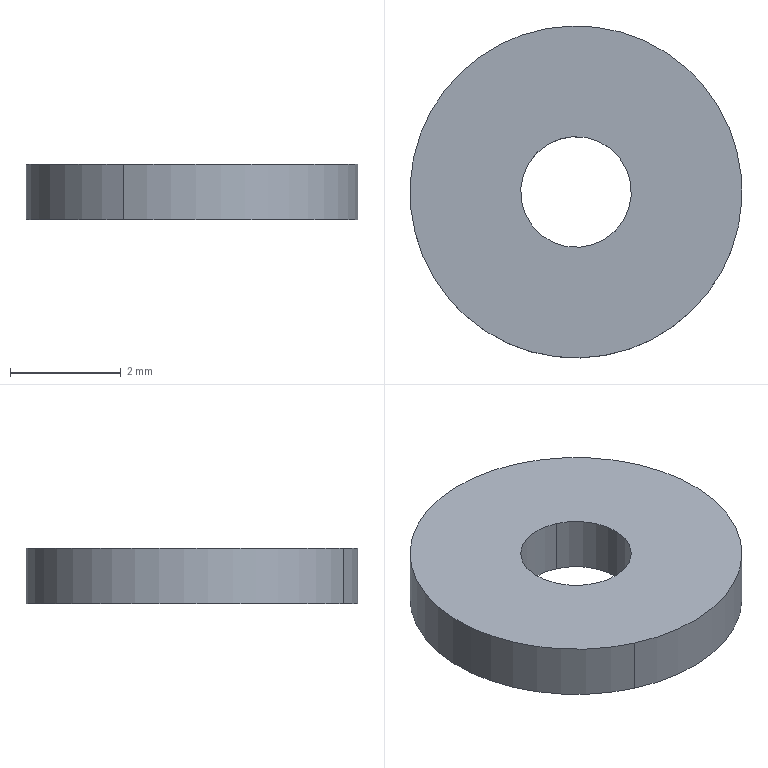Component | SolidWorks | Part28^Assembly1-2 | 1 solid | 6 faces | box 6 x 6 x 1 mm | volume 25 mm3 | cylinder 4 | plane 2 | commonest cylinder face diameters 2 x2 6 x2
STEP:
#1=COLOUR_RGB('',0.7922,0.8196,0.9333);
#2=FILL_AREA_STYLE_COLOUR('',#1);
#3=FILL_AREA_STYLE('',(#2));
#4=SURFACE_STYLE_FILL_AREA(#3);
#5=SURFACE_SIDE_STYLE('',(#4));
#6=SURFACE_STYLE_USAGE(.BOTH.,#5);
#7=PRESENTATION_STYLE_ASSIGNMENT((#6));
#8=CARTESIAN_POINT('',(0.5083,-0.1019,0.1575));
#9=VERTEX_POINT('',#8);
#10=CARTESIAN_POINT('',(0.4759,-0.1737,0.1575));
#11=VERTEX_POINT('',#10);
#12=CARTESIAN_POINT('',(0.4921,-0.1378,0.1575));
#13=DIRECTION('',(-0.,-0.,1.));
#14=DIRECTION('',(-0.412,-0.9112,-0.));
#15=AXIS2_PLACEMENT_3D('',#12,#13,#14);
#16=CIRCLE('',#15,0.03937);
#17=EDGE_CURVE('',#9,#11,#16,.T.);
#18=ORIENTED_EDGE('',*,*,#17,.T.);
#19=CARTESIAN_POINT('',(0.4759,-0.1737,0.1181));
#20=VERTEX_POINT('',#19);
#21=CARTESIAN_POINT('',(0.4759,-0.1737,0.1575));
#22=DIRECTION('',(0.,0.,-1.));
#23=VECTOR('',#22,39.37);
#24=LINE('',#21,#23);
#25=EDGE_CURVE('',#11,#20,#24,.T.);
#26=ORIENTED_EDGE('',*,*,#25,.T.);
#27=CARTESIAN_POINT('',(0.5083,-0.1019,0.1181));
#28=VERTEX_POINT('',#27);
#29=CARTESIAN_POINT('',(0.4921,-0.1378,0.1181));
#30=DIRECTION('',(-0.,-0.,1.));
#31=DIRECTION('',(-0.412,-0.9112,-0.));
#32=AXIS2_PLACEMENT_3D('',#29,#30,#31);
#33=CIRCLE('',#32,0.03937);
#34=EDGE_CURVE('',#28,#20,#33,.T.);
#35=ORIENTED_EDGE('',*,*,#34,.F.);
#36=CARTESIAN_POINT('',(0.5083,-0.1019,0.1575));
#37=DIRECTION('',(0.,0.,-1.));
#38=VECTOR('',#37,39.37);
#39=LINE('',#36,#38);
#40=EDGE_CURVE('',#9,#28,#39,.T.);
#41=ORIENTED_EDGE('',*,*,#40,.F.);
#42=EDGE_LOOP('',(#18,#26,#35,#41));
#43=FACE_OUTER_BOUND('',#42,.T.);
#44=CARTESIAN_POINT('',(0.4921,-0.1378,0.1575));
#45=DIRECTION('',(0.,0.,-1.));
#46=DIRECTION('',(0.412,0.9112,0.));
#47=AXIS2_PLACEMENT_3D('',#44,#45,#46);
#48=CYLINDRICAL_SURFACE('',#47,0.03937);
#49=ADVANCED_FACE('',(#43),#48,.F.);
#50=CARTESIAN_POINT('',(0.4435,-0.2454,0.1575));
#51=VERTEX_POINT('',#50);
#52=CARTESIAN_POINT('',(0.5408,-0.03017,0.1575));
#53=VERTEX_POINT('',#52);
#54=CARTESIAN_POINT('',(0.4921,-0.1378,0.1575));
#55=DIRECTION('',(-0.,-0.,1.));
#56=DIRECTION('',(-0.412,-0.9112,-0.));
#57=AXIS2_PLACEMENT_3D('',#54,#55,#56);
#58=CIRCLE('',#57,0.1181);
#59=EDGE_CURVE('',#51,#53,#58,.T.);
#60=ORIENTED_EDGE('',*,*,#59,.F.);
#61=CARTESIAN_POINT('',(0.4435,-0.2454,0.1181));
#62=VERTEX_POINT('',#61);
#63=CARTESIAN_POINT('',(0.4435,-0.2454,0.1575));
#64=DIRECTION('',(0.,0.,-1.));
#65=VECTOR('',#64,39.37);
#66=LINE('',#63,#65);
#67=EDGE_CURVE('',#51,#62,#66,.T.);
#68=ORIENTED_EDGE('',*,*,#67,.T.);
#69=CARTESIAN_POINT('',(0.5408,-0.03017,0.1181));
#70=VERTEX_POINT('',#69);
#71=CARTESIAN_POINT('',(0.4921,-0.1378,0.1181));
#72=DIRECTION('',(-0.,-0.,1.));
#73=DIRECTION('',(-0.412,-0.9112,-0.));
#74=AXIS2_PLACEMENT_3D('',#71,#72,#73);
#75=CIRCLE('',#74,0.1181);
#76=EDGE_CURVE('',#62,#70,#75,.T.);
#77=ORIENTED_EDGE('',*,*,#76,.T.);
#78=CARTESIAN_POINT('',(0.5408,-0.03017,0.1575));
#79=DIRECTION('',(0.,0.,-1.));
#80=VECTOR('',#79,39.37);
#81=LINE('',#78,#80);
#82=EDGE_CURVE('',#53,#70,#81,.T.);
#83=ORIENTED_EDGE('',*,*,#82,.F.);
#84=EDGE_LOOP('',(#60,#68,#77,#83));
#85=FACE_OUTER_BOUND('',#84,.T.);
#86=CARTESIAN_POINT('',(0.4921,-0.1378,0.1575));
#87=DIRECTION('',(0.,0.,-1.));
#88=DIRECTION('',(0.412,0.9112,0.));
#89=AXIS2_PLACEMENT_3D('',#86,#87,#88);
#90=CYLINDRICAL_SURFACE('',#89,0.1181);
#91=ADVANCED_FACE('',(#85),#90,.T.);
#92=CARTESIAN_POINT('',(0.4921,-0.1378,0.1575));
#93=DIRECTION('',(-0.,-0.,1.));
#94=DIRECTION('',(-0.412,-0.9112,-0.));
#95=AXIS2_PLACEMENT_3D('',#92,#93,#94);
#96=CIRCLE('',#95,0.1181);
#97=EDGE_CURVE('',#53,#51,#96,.T.);
#98=ORIENTED_EDGE('',*,*,#97,.T.);
#99=ORIENTED_EDGE('',*,*,#59,.T.);
#100=EDGE_LOOP('',(#98,#99));
#101=FACE_OUTER_BOUND('',#100,.T.);
#102=ORIENTED_EDGE('',*,*,#17,.F.);
#103=CARTESIAN_POINT('',(0.4921,-0.1378,0.1575));
#104=DIRECTION('',(-0.,-0.,1.));
#105=DIRECTION('',(-0.412,-0.9112,-0.));
#106=AXIS2_PLACEMENT_3D('',#103,#104,#105);
#107=CIRCLE('',#106,0.03937);
#108=EDGE_CURVE('',#11,#9,#107,.T.);
#109=ORIENTED_EDGE('',*,*,#108,.F.);
#110=EDGE_LOOP('',(#102,#109));
#111=FACE_BOUND('',#110,.T.);
#112=CARTESIAN_POINT('',(0.4921,-0.1378,0.1575));
#113=DIRECTION('',(-0.,-0.,1.));
#114=DIRECTION('',(-0.412,-0.9112,-0.));
#115=AXIS2_PLACEMENT_3D('',#112,#113,#114);
#116=PLANE('',#115);
#117=ADVANCED_FACE('',(#101,#111),#116,.T.);
#118=CARTESIAN_POINT('',(0.4921,-0.1378,0.1181));
#119=DIRECTION('',(-0.,-0.,1.));
#120=DIRECTION('',(-0.412,-0.9112,-0.));
#121=AXIS2_PLACEMENT_3D('',#118,#119,#120);
#122=CIRCLE('',#121,0.1181);
#123=EDGE_CURVE('',#70,#62,#122,.T.);
#124=ORIENTED_EDGE('',*,*,#123,.F.);
#125=ORIENTED_EDGE('',*,*,#76,.F.);
#126=EDGE_LOOP('',(#124,#125));
#127=FACE_OUTER_BOUND('',#126,.T.);
#128=ORIENTED_EDGE('',*,*,#34,.T.);
#129=CARTESIAN_POINT('',(0.4921,-0.1378,0.1181));
#130=DIRECTION('',(-0.,-0.,1.));
#131=DIRECTION('',(-0.412,-0.9112,-0.));
#132=AXIS2_PLACEMENT_3D('',#129,#130,#131);
#133=CIRCLE('',#132,0.03937);
#134=EDGE_CURVE('',#20,#28,#133,.T.);
#135=ORIENTED_EDGE('',*,*,#134,.T.);
#136=EDGE_LOOP('',(#128,#135));
#137=FACE_BOUND('',#136,.T.);
#138=CARTESIAN_POINT('',(0.4921,-0.1378,0.1181));
#139=DIRECTION('',(-0.,-0.,1.));
#140=DIRECTION('',(-0.412,-0.9112,-0.));
#141=AXIS2_PLACEMENT_3D('',#138,#139,#140);
#142=PLANE('',#141);
#143=ADVANCED_FACE('',(#127,#137),#142,.F.);
#144=ORIENTED_EDGE('',*,*,#67,.F.);
#145=ORIENTED_EDGE('',*,*,#97,.F.);
#146=ORIENTED_EDGE('',*,*,#82,.T.);
#147=ORIENTED_EDGE('',*,*,#123,.T.);
#148=EDGE_LOOP('',(#144,#145,#146,#147));
#149=FACE_OUTER_BOUND('',#148,.T.);
#150=CARTESIAN_POINT('',(0.4921,-0.1378,0.1575));
#151=DIRECTION('',(0.,0.,-1.));
#152=DIRECTION('',(0.412,0.9112,0.));
#153=AXIS2_PLACEMENT_3D('',#150,#151,#152);
#154=CYLINDRICAL_SURFACE('',#153,0.1181);
#155=ADVANCED_FACE('',(#149),#154,.T.);
#156=ORIENTED_EDGE('',*,*,#25,.F.);
#157=ORIENTED_EDGE('',*,*,#108,.T.);
#158=ORIENTED_EDGE('',*,*,#40,.T.);
#159=ORIENTED_EDGE('',*,*,#134,.F.);
#160=EDGE_LOOP('',(#156,#157,#158,#159));
#161=FACE_OUTER_BOUND('',#160,.T.);
#162=CARTESIAN_POINT('',(0.4921,-0.1378,0.1575));
#163=DIRECTION('',(0.,0.,-1.));
#164=DIRECTION('',(0.412,0.9112,0.));
#165=AXIS2_PLACEMENT_3D('',#162,#163,#164);
#166=CYLINDRICAL_SURFACE('',#165,0.03937);
#167=ADVANCED_FACE('',(#161),#166,.F.);
#168=CLOSED_SHELL('',(#49,#91,#117,#143,#155,#167));
#169=MANIFOLD_SOLID_BREP('',#168);
#170=STYLED_ITEM('',(#7),#169);
#171=(LENGTH_UNIT()NAMED_UNIT(*)SI_UNIT($,.METRE.));
#172=LENGTH_MEASURE_WITH_UNIT(LENGTH_MEASURE(0.0254),#171);
#173=DIMENSIONAL_EXPONENTS(1.,0.,0.,0.,0.,0.,0.);
#174=(CONVERSION_BASED_UNIT('',#172)LENGTH_UNIT()NAMED_UNIT(#173));
#175=UNCERTAINTY_MEASURE_WITH_UNIT(LENGTH_MEASURE(0.00001),#174,'','');
#176=(NAMED_UNIT(*)PLANE_ANGLE_UNIT()SI_UNIT($,.RADIAN.));
#177=(NAMED_UNIT(*)SI_UNIT($,.STERADIAN.)SOLID_ANGLE_UNIT());
#178=(GEOMETRIC_REPRESENTATION_CONTEXT(3)GLOBAL_UNCERTAINTY_ASSIGNED_CONTEXT((#175))GLOBAL_UNIT_ASSIGNED_CONTEXT((#174,#176,#177))REPRESENTATION_CONTEXT('',''));
#179=MECHANICAL_DESIGN_GEOMETRIC_PRESENTATION_REPRESENTATION('',(#170),#178);
#180=PRESENTATION_LAYER_ASSIGNMENT('','',(#170));
#181=CARTESIAN_POINT('',(0.,0.,0.));
#182=DIRECTION('',(0.,0.,1.));
#183=DIRECTION('',(1.,0.,0.));
#184=AXIS2_PLACEMENT_3D('',#181,#182,#183);
#185=(LENGTH_UNIT()NAMED_UNIT(*)SI_UNIT($,.METRE.));
#186=LENGTH_MEASURE_WITH_UNIT(LENGTH_MEASURE(0.0254),#185);
#187=DIMENSIONAL_EXPONENTS(1.,0.,0.,0.,0.,0.,0.);
#188=(CONVERSION_BASED_UNIT('',#186)LENGTH_UNIT()NAMED_UNIT(#187));
#189=UNCERTAINTY_MEASURE_WITH_UNIT(LENGTH_MEASURE(0.00001),#188,'','');
#190=(NAMED_UNIT(*)PLANE_ANGLE_UNIT()SI_UNIT($,.RADIAN.));
#191=(NAMED_UNIT(*)SI_UNIT($,.STERADIAN.)SOLID_ANGLE_UNIT());
#192=(GEOMETRIC_REPRESENTATION_CONTEXT(3)GLOBAL_UNCERTAINTY_ASSIGNED_CONTEXT((#189))GLOBAL_UNIT_ASSIGNED_CONTEXT((#188,#190,#191))REPRESENTATION_CONTEXT('',''));
#193=ADVANCED_BREP_SHAPE_REPRESENTATION('',(#169,#184),#192);